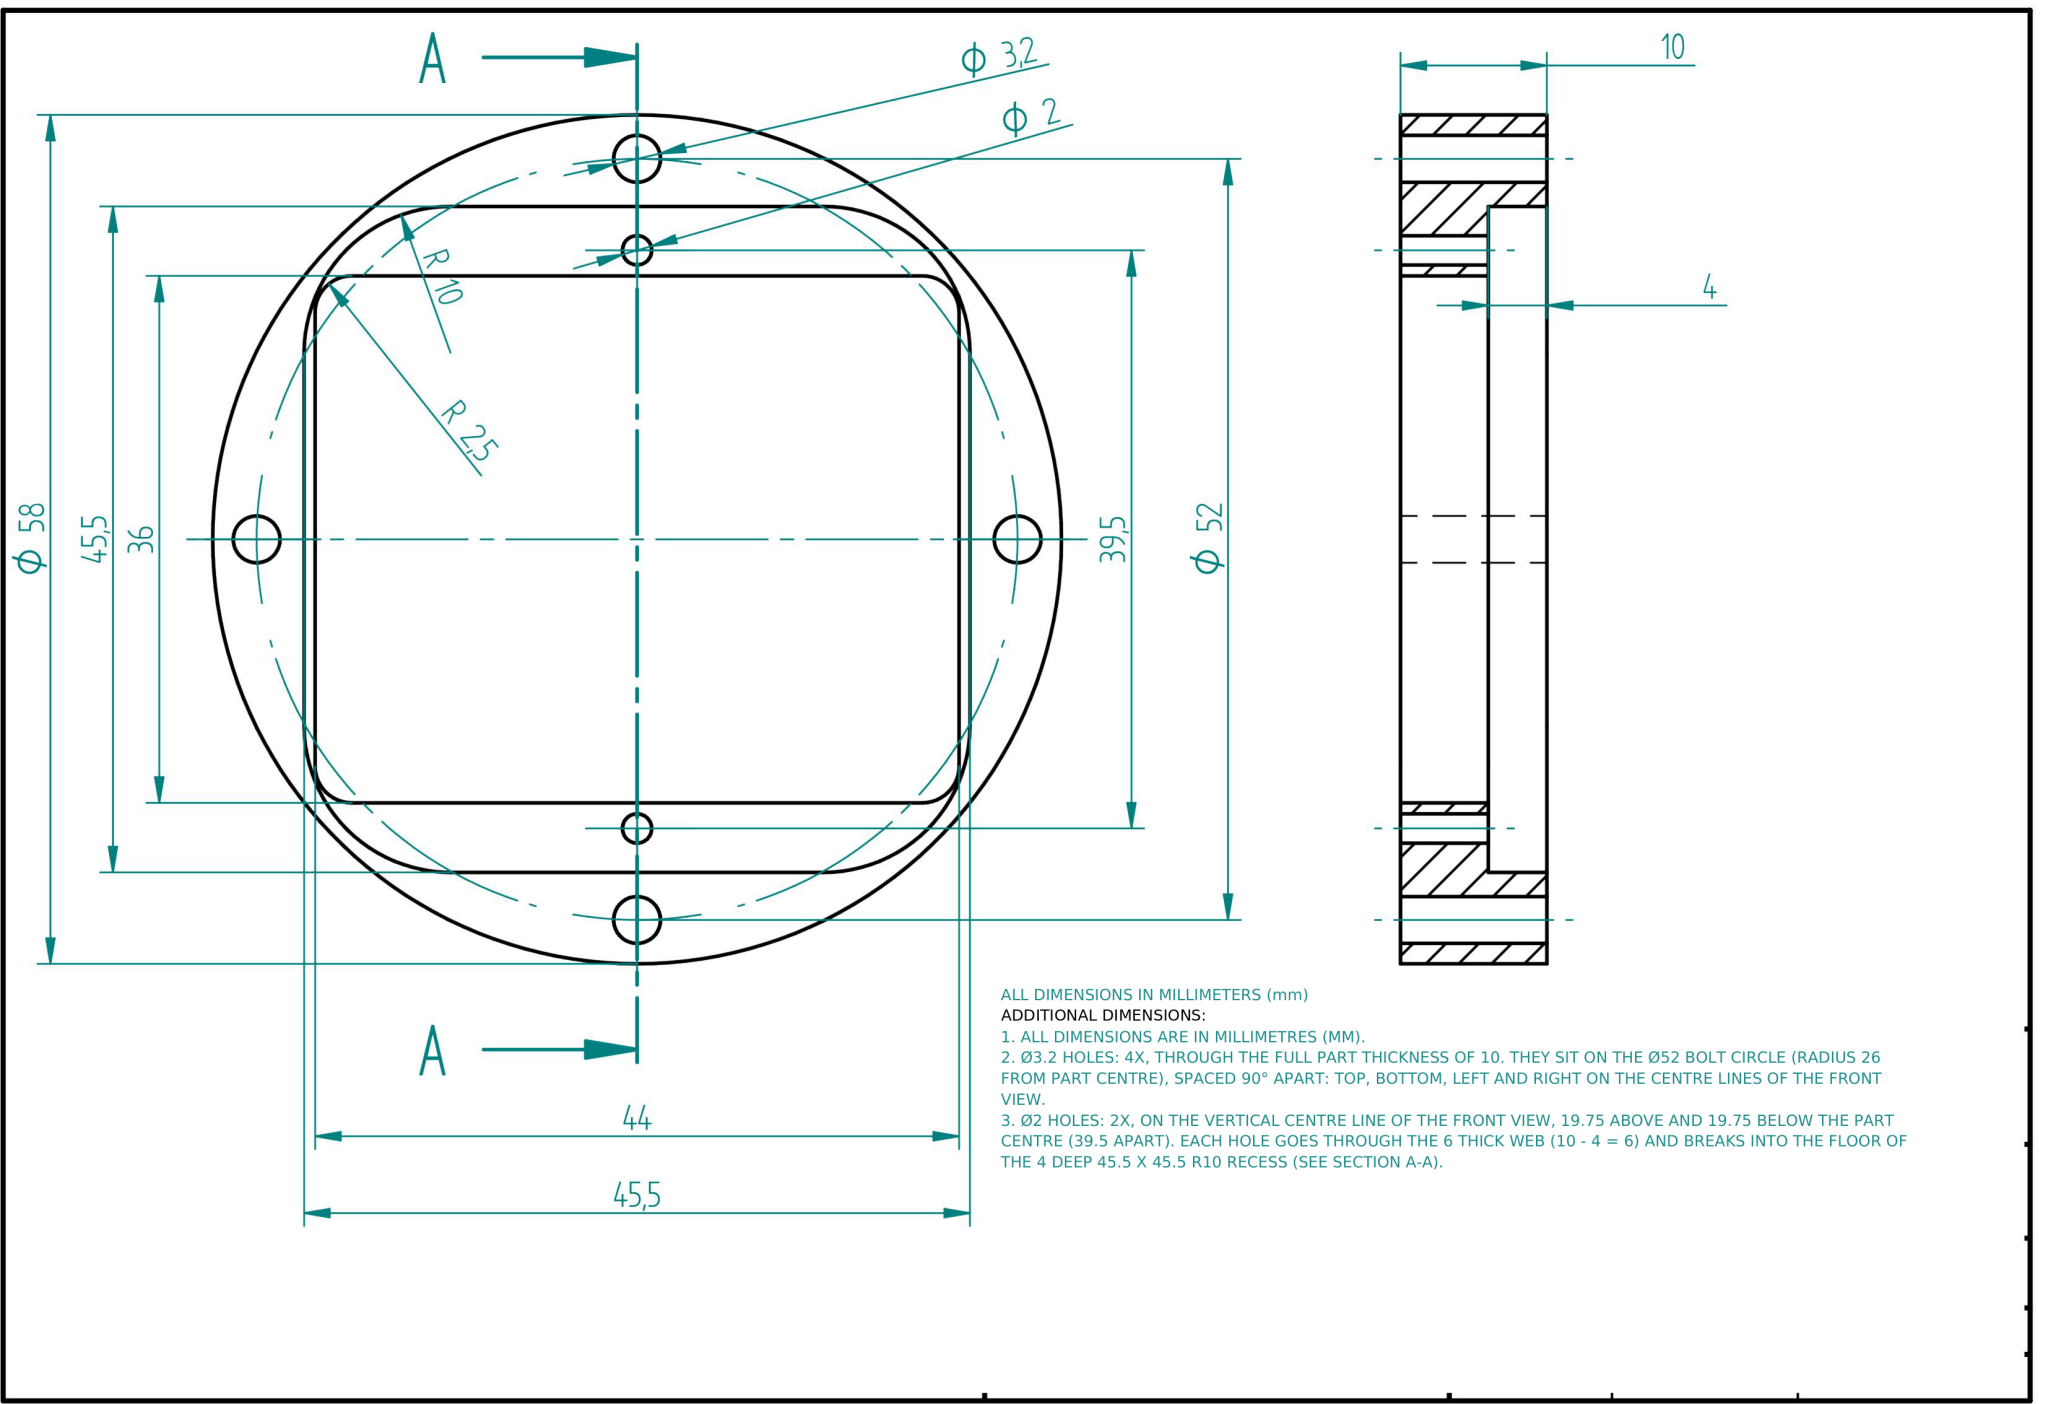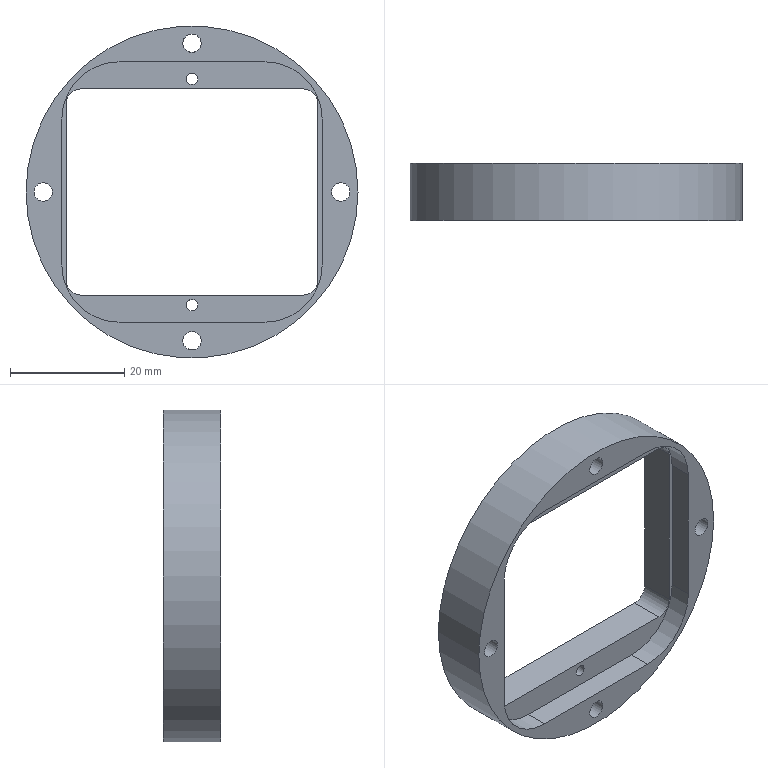Part | NX | mm | Triangular Flanged Gasket Ring | 1 solid | 26 faces | box 58 x 10 x 58 mm | volume 8652 mm3 | cylinder 15 | plane 11 | commonest cylinder face diameters 20 x4 5 x4 3.2 x4 2 x2 58 x1
STEP:
#1=COLOUR_RGB('',0.,0.698,0.);
#2=FILL_AREA_STYLE_COLOUR('',#1);
#3=FILL_AREA_STYLE('',(#2));
#4=SURFACE_STYLE_FILL_AREA(#3);
#5=SURFACE_SIDE_STYLE('',(#4));
#6=SURFACE_STYLE_USAGE(.BOTH.,#5);
#7=PRESENTATION_STYLE_ASSIGNMENT((#6));
#8=CARTESIAN_POINT('',(-26.,0.,1.6));
#9=VERTEX_POINT('',#8);
#10=CARTESIAN_POINT('',(-26.,0.,-0.));
#11=DIRECTION('',(0.,-1.,0.));
#12=DIRECTION('',(-0.,0.,1.));
#13=AXIS2_PLACEMENT_3D('',#10,#11,#12);
#14=CIRCLE('',#13,1.6);
#15=EDGE_CURVE('',#9,#9,#14,.T.);
#16=ORIENTED_EDGE('',*,*,#15,.F.);
#17=EDGE_LOOP('',(#16));
#18=FACE_BOUND('',#17,.T.);
#19=CARTESIAN_POINT('',(-1.6,0.,-26.));
#20=VERTEX_POINT('',#19);
#21=CARTESIAN_POINT('',(-0.,0.,-26.));
#22=DIRECTION('',(0.,-1.,0.));
#23=DIRECTION('',(-1.,0.,0.));
#24=AXIS2_PLACEMENT_3D('',#21,#22,#23);
#25=CIRCLE('',#24,1.6);
#26=EDGE_CURVE('',#20,#20,#25,.T.);
#27=ORIENTED_EDGE('',*,*,#26,.F.);
#28=EDGE_LOOP('',(#27));
#29=FACE_BOUND('',#28,.T.);
#30=CARTESIAN_POINT('',(26.,0.,-1.6));
#31=VERTEX_POINT('',#30);
#32=CARTESIAN_POINT('',(26.,0.,-0.));
#33=DIRECTION('',(0.,-1.,0.));
#34=DIRECTION('',(-0.,0.,-1.));
#35=AXIS2_PLACEMENT_3D('',#32,#33,#34);
#36=CIRCLE('',#35,1.6);
#37=EDGE_CURVE('',#31,#31,#36,.T.);
#38=ORIENTED_EDGE('',*,*,#37,.F.);
#39=EDGE_LOOP('',(#38));
#40=FACE_BOUND('',#39,.T.);
#41=CARTESIAN_POINT('',(1.6,0.,26.));
#42=VERTEX_POINT('',#41);
#43=CARTESIAN_POINT('',(0.,0.,26.));
#44=DIRECTION('',(0.,-1.,0.));
#45=DIRECTION('',(1.,0.,0.));
#46=AXIS2_PLACEMENT_3D('',#43,#44,#45);
#47=CIRCLE('',#46,1.6);
#48=EDGE_CURVE('',#42,#42,#47,.T.);
#49=ORIENTED_EDGE('',*,*,#48,.F.);
#50=EDGE_LOOP('',(#49));
#51=FACE_BOUND('',#50,.T.);
#52=CARTESIAN_POINT('',(29.,0.,0.));
#53=VERTEX_POINT('',#52);
#54=CARTESIAN_POINT('',(0.,0.,0.));
#55=DIRECTION('',(0.,1.,0.));
#56=DIRECTION('',(1.,0.,0.));
#57=AXIS2_PLACEMENT_3D('',#54,#55,#56);
#58=CIRCLE('',#57,29.);
#59=EDGE_CURVE('',#53,#53,#58,.T.);
#60=ORIENTED_EDGE('',*,*,#59,.F.);
#61=EDGE_LOOP('',(#60));
#62=FACE_OUTER_BOUND('',#61,.T.);
#63=CARTESIAN_POINT('',(22.75,0.,-12.75));
#64=VERTEX_POINT('',#63);
#65=CARTESIAN_POINT('',(12.75,0.,-22.75));
#66=VERTEX_POINT('',#65);
#67=CARTESIAN_POINT('',(12.75,0.,-12.75));
#68=DIRECTION('',(0.,1.,0.));
#69=DIRECTION('',(-1.,0.,0.));
#70=AXIS2_PLACEMENT_3D('',#67,#68,#69);
#71=CIRCLE('',#70,10.);
#72=EDGE_CURVE('',#64,#66,#71,.T.);
#73=ORIENTED_EDGE('',*,*,#72,.T.);
#74=CARTESIAN_POINT('',(-12.75,0.,-22.75));
#75=VERTEX_POINT('',#74);
#76=CARTESIAN_POINT('',(22.75,0.,-22.75));
#77=DIRECTION('',(-1.,0.,-0.));
#78=VECTOR('',#77,1000.);
#79=LINE('',#76,#78);
#80=EDGE_CURVE('',#66,#75,#79,.T.);
#81=ORIENTED_EDGE('',*,*,#80,.T.);
#82=CARTESIAN_POINT('',(-22.75,0.,-12.75));
#83=VERTEX_POINT('',#82);
#84=CARTESIAN_POINT('',(-12.75,0.,-12.75));
#85=DIRECTION('',(0.,1.,0.));
#86=DIRECTION('',(1.,0.,0.));
#87=AXIS2_PLACEMENT_3D('',#84,#85,#86);
#88=CIRCLE('',#87,10.);
#89=EDGE_CURVE('',#75,#83,#88,.T.);
#90=ORIENTED_EDGE('',*,*,#89,.T.);
#91=CARTESIAN_POINT('',(-22.75,0.,12.75));
#92=VERTEX_POINT('',#91);
#93=CARTESIAN_POINT('',(-22.75,0.,-22.75));
#94=DIRECTION('',(-0.,0.,1.));
#95=VECTOR('',#94,1000.);
#96=LINE('',#93,#95);
#97=EDGE_CURVE('',#83,#92,#96,.T.);
#98=ORIENTED_EDGE('',*,*,#97,.T.);
#99=CARTESIAN_POINT('',(-12.75,0.,22.75));
#100=VERTEX_POINT('',#99);
#101=CARTESIAN_POINT('',(-12.75,0.,12.75));
#102=DIRECTION('',(0.,1.,0.));
#103=DIRECTION('',(1.,0.,0.));
#104=AXIS2_PLACEMENT_3D('',#101,#102,#103);
#105=CIRCLE('',#104,10.);
#106=EDGE_CURVE('',#92,#100,#105,.T.);
#107=ORIENTED_EDGE('',*,*,#106,.T.);
#108=CARTESIAN_POINT('',(12.75,0.,22.75));
#109=VERTEX_POINT('',#108);
#110=CARTESIAN_POINT('',(-22.75,0.,22.75));
#111=DIRECTION('',(1.,0.,0.));
#112=VECTOR('',#111,1000.);
#113=LINE('',#110,#112);
#114=EDGE_CURVE('',#100,#109,#113,.T.);
#115=ORIENTED_EDGE('',*,*,#114,.T.);
#116=CARTESIAN_POINT('',(22.75,0.,12.75));
#117=VERTEX_POINT('',#116);
#118=CARTESIAN_POINT('',(12.75,0.,12.75));
#119=DIRECTION('',(0.,1.,0.));
#120=DIRECTION('',(-1.,0.,0.));
#121=AXIS2_PLACEMENT_3D('',#118,#119,#120);
#122=CIRCLE('',#121,10.);
#123=EDGE_CURVE('',#109,#117,#122,.T.);
#124=ORIENTED_EDGE('',*,*,#123,.T.);
#125=CARTESIAN_POINT('',(22.75,0.,22.75));
#126=DIRECTION('',(0.,0.,-1.));
#127=VECTOR('',#126,1000.);
#128=LINE('',#125,#127);
#129=EDGE_CURVE('',#117,#64,#128,.T.);
#130=ORIENTED_EDGE('',*,*,#129,.T.);
#131=EDGE_LOOP('',(#73,#81,#90,#98,#107,#115,#124,#130));
#132=FACE_BOUND('',#131,.T.);
#133=CARTESIAN_POINT('',(0.,0.,0.));
#134=DIRECTION('',(0.,1.,0.));
#135=DIRECTION('',(0.,0.,1.));
#136=AXIS2_PLACEMENT_3D('',#133,#134,#135);
#137=PLANE('',#136);
#138=ADVANCED_FACE('',(#18,#29,#40,#51,#62,#132),#137,.F.);
#139=STYLED_ITEM('',(#7),#138);
#140=COLOUR_RGB('',0.,0.698,0.);
#141=FILL_AREA_STYLE_COLOUR('',#140);
#142=FILL_AREA_STYLE('',(#141));
#143=SURFACE_STYLE_FILL_AREA(#142);
#144=SURFACE_SIDE_STYLE('',(#143));
#145=SURFACE_STYLE_USAGE(.BOTH.,#144);
#146=PRESENTATION_STYLE_ASSIGNMENT((#145));
#147=ORIENTED_EDGE('',*,*,#80,.F.);
#148=CARTESIAN_POINT('',(12.75,4.,-22.75));
#149=VERTEX_POINT('',#148);
#150=CARTESIAN_POINT('',(12.75,4.,-22.75));
#151=DIRECTION('',(0.,-1.,0.));
#152=VECTOR('',#151,1000.);
#153=LINE('',#150,#152);
#154=EDGE_CURVE('',#149,#66,#153,.T.);
#155=ORIENTED_EDGE('',*,*,#154,.F.);
#156=CARTESIAN_POINT('',(-12.75,4.,-22.75));
#157=VERTEX_POINT('',#156);
#158=CARTESIAN_POINT('',(22.75,4.,-22.75));
#159=DIRECTION('',(-1.,0.,-0.));
#160=VECTOR('',#159,1000.);
#161=LINE('',#158,#160);
#162=EDGE_CURVE('',#149,#157,#161,.T.);
#163=ORIENTED_EDGE('',*,*,#162,.T.);
#164=CARTESIAN_POINT('',(-12.75,4.,-22.75));
#165=DIRECTION('',(0.,-1.,0.));
#166=VECTOR('',#165,1000.);
#167=LINE('',#164,#166);
#168=EDGE_CURVE('',#157,#75,#167,.T.);
#169=ORIENTED_EDGE('',*,*,#168,.T.);
#170=EDGE_LOOP('',(#147,#155,#163,#169));
#171=FACE_OUTER_BOUND('',#170,.T.);
#172=CARTESIAN_POINT('',(22.75,4.,-22.75));
#173=DIRECTION('',(-0.,0.,1.));
#174=DIRECTION('',(1.,0.,0.));
#175=AXIS2_PLACEMENT_3D('',#172,#173,#174);
#176=PLANE('',#175);
#177=ADVANCED_FACE('',(#171),#176,.T.);
#178=STYLED_ITEM('',(#146),#177);
#179=COLOUR_RGB('',0.,0.698,0.);
#180=FILL_AREA_STYLE_COLOUR('',#179);
#181=FILL_AREA_STYLE('',(#180));
#182=SURFACE_STYLE_FILL_AREA(#181);
#183=SURFACE_SIDE_STYLE('',(#182));
#184=SURFACE_STYLE_USAGE(.BOTH.,#183);
#185=PRESENTATION_STYLE_ASSIGNMENT((#184));
#186=CARTESIAN_POINT('',(19.5,4.,-18.));
#187=VERTEX_POINT('',#186);
#188=CARTESIAN_POINT('',(-19.5,4.,-18.));
#189=VERTEX_POINT('',#188);
#190=CARTESIAN_POINT('',(22.,4.,-18.));
#191=DIRECTION('',(-1.,0.,0.));
#192=VECTOR('',#191,1000.);
#193=LINE('',#190,#192);
#194=EDGE_CURVE('',#187,#189,#193,.T.);
#195=ORIENTED_EDGE('',*,*,#194,.F.);
#196=CARTESIAN_POINT('',(19.5,10.,-18.));
#197=VERTEX_POINT('',#196);
#198=CARTESIAN_POINT('',(19.5,84.,-18.));
#199=DIRECTION('',(0.,-1.,0.));
#200=VECTOR('',#199,1000.);
#201=LINE('',#198,#200);
#202=EDGE_CURVE('',#197,#187,#201,.T.);
#203=ORIENTED_EDGE('',*,*,#202,.F.);
#204=CARTESIAN_POINT('',(-19.5,10.,-18.));
#205=VERTEX_POINT('',#204);
#206=CARTESIAN_POINT('',(0.,10.,-18.));
#207=DIRECTION('',(1.,0.,0.));
#208=VECTOR('',#207,1000.);
#209=LINE('',#206,#208);
#210=EDGE_CURVE('',#205,#197,#209,.T.);
#211=ORIENTED_EDGE('',*,*,#210,.F.);
#212=CARTESIAN_POINT('',(-19.5,84.,-18.));
#213=DIRECTION('',(0.,-1.,0.));
#214=VECTOR('',#213,1000.);
#215=LINE('',#212,#214);
#216=EDGE_CURVE('',#205,#189,#215,.T.);
#217=ORIENTED_EDGE('',*,*,#216,.T.);
#218=EDGE_LOOP('',(#195,#203,#211,#217));
#219=FACE_OUTER_BOUND('',#218,.T.);
#220=CARTESIAN_POINT('',(22.,84.,-18.));
#221=DIRECTION('',(0.,0.,1.));
#222=DIRECTION('',(1.,0.,0.));
#223=AXIS2_PLACEMENT_3D('',#220,#221,#222);
#224=PLANE('',#223);
#225=ADVANCED_FACE('',(#219),#224,.T.);
#226=STYLED_ITEM('',(#185),#225);
#227=COLOUR_RGB('',0.,0.698,0.);
#228=FILL_AREA_STYLE_COLOUR('',#227);
#229=FILL_AREA_STYLE('',(#228));
#230=SURFACE_STYLE_FILL_AREA(#229);
#231=SURFACE_SIDE_STYLE('',(#230));
#232=SURFACE_STYLE_USAGE(.BOTH.,#231);
#233=PRESENTATION_STYLE_ASSIGNMENT((#232));
#234=CARTESIAN_POINT('',(0.,10.,-18.75));
#235=VERTEX_POINT('',#234);
#236=CARTESIAN_POINT('',(0.,10.,-19.75));
#237=DIRECTION('',(0.,1.,0.));
#238=DIRECTION('',(0.,0.,1.));
#239=AXIS2_PLACEMENT_3D('',#236,#237,#238);
#240=CIRCLE('',#239,1.);
#241=EDGE_CURVE('',#235,#235,#240,.T.);
#242=ORIENTED_EDGE('',*,*,#241,.F.);
#243=EDGE_LOOP('',(#242));
#244=FACE_BOUND('',#243,.T.);
#245=CARTESIAN_POINT('',(0.,10.,20.75));
#246=VERTEX_POINT('',#245);
#247=CARTESIAN_POINT('',(0.,10.,19.75));
#248=DIRECTION('',(0.,1.,0.));
#249=DIRECTION('',(0.,0.,1.));
#250=AXIS2_PLACEMENT_3D('',#247,#248,#249);
#251=CIRCLE('',#250,1.);
#252=EDGE_CURVE('',#246,#246,#251,.T.);
#253=ORIENTED_EDGE('',*,*,#252,.F.);
#254=EDGE_LOOP('',(#253));
#255=FACE_BOUND('',#254,.T.);
#256=CARTESIAN_POINT('',(-26.,10.,1.6));
#257=VERTEX_POINT('',#256);
#258=CARTESIAN_POINT('',(-26.,10.,-0.));
#259=DIRECTION('',(0.,1.,0.));
#260=DIRECTION('',(0.,0.,1.));
#261=AXIS2_PLACEMENT_3D('',#258,#259,#260);
#262=CIRCLE('',#261,1.6);
#263=EDGE_CURVE('',#257,#257,#262,.T.);
#264=ORIENTED_EDGE('',*,*,#263,.F.);
#265=EDGE_LOOP('',(#264));
#266=FACE_BOUND('',#265,.T.);
#267=CARTESIAN_POINT('',(-0.,10.,-24.4));
#268=VERTEX_POINT('',#267);
#269=CARTESIAN_POINT('',(-0.,10.,-26.));
#270=DIRECTION('',(0.,1.,0.));
#271=DIRECTION('',(0.,0.,1.));
#272=AXIS2_PLACEMENT_3D('',#269,#270,#271);
#273=CIRCLE('',#272,1.6);
#274=EDGE_CURVE('',#268,#268,#273,.T.);
#275=ORIENTED_EDGE('',*,*,#274,.F.);
#276=EDGE_LOOP('',(#275));
#277=FACE_BOUND('',#276,.T.);
#278=CARTESIAN_POINT('',(26.,10.,1.6));
#279=VERTEX_POINT('',#278);
#280=CARTESIAN_POINT('',(26.,10.,-0.));
#281=DIRECTION('',(0.,1.,0.));
#282=DIRECTION('',(0.,0.,1.));
#283=AXIS2_PLACEMENT_3D('',#280,#281,#282);
#284=CIRCLE('',#283,1.6);
#285=EDGE_CURVE('',#279,#279,#284,.T.);
#286=ORIENTED_EDGE('',*,*,#285,.F.);
#287=EDGE_LOOP('',(#286));
#288=FACE_BOUND('',#287,.T.);
#289=CARTESIAN_POINT('',(0.,10.,27.6));
#290=VERTEX_POINT('',#289);
#291=CARTESIAN_POINT('',(0.,10.,26.));
#292=DIRECTION('',(0.,1.,0.));
#293=DIRECTION('',(0.,0.,1.));
#294=AXIS2_PLACEMENT_3D('',#291,#292,#293);
#295=CIRCLE('',#294,1.6);
#296=EDGE_CURVE('',#290,#290,#295,.T.);
#297=ORIENTED_EDGE('',*,*,#296,.F.);
#298=EDGE_LOOP('',(#297));
#299=FACE_BOUND('',#298,.T.);
#300=CARTESIAN_POINT('',(29.,10.,0.));
#301=VERTEX_POINT('',#300);
#302=CARTESIAN_POINT('',(0.,10.,0.));
#303=DIRECTION('',(0.,1.,0.));
#304=DIRECTION('',(1.,0.,0.));
#305=AXIS2_PLACEMENT_3D('',#302,#303,#304);
#306=CIRCLE('',#305,29.);
#307=EDGE_CURVE('',#301,#301,#306,.T.);
#308=ORIENTED_EDGE('',*,*,#307,.T.);
#309=EDGE_LOOP('',(#308));
#310=FACE_OUTER_BOUND('',#309,.T.);
#311=CARTESIAN_POINT('',(19.5,10.,18.));
#312=VERTEX_POINT('',#311);
#313=CARTESIAN_POINT('',(-19.5,10.,18.));
#314=VERTEX_POINT('',#313);
#315=CARTESIAN_POINT('',(0.,10.,18.));
#316=DIRECTION('',(-1.,0.,0.));
#317=VECTOR('',#316,1000.);
#318=LINE('',#315,#317);
#319=EDGE_CURVE('',#312,#314,#318,.T.);
#320=ORIENTED_EDGE('',*,*,#319,.T.);
#321=CARTESIAN_POINT('',(-22.,10.,15.5));
#322=VERTEX_POINT('',#321);
#323=CARTESIAN_POINT('',(-19.5,10.,15.5));
#324=DIRECTION('',(0.,1.,0.));
#325=DIRECTION('',(0.,0.,1.));
#326=AXIS2_PLACEMENT_3D('',#323,#324,#325);
#327=CIRCLE('',#326,2.5);
#328=EDGE_CURVE('',#314,#322,#327,.F.);
#329=ORIENTED_EDGE('',*,*,#328,.T.);
#330=CARTESIAN_POINT('',(-22.,10.,-15.5));
#331=VERTEX_POINT('',#330);
#332=CARTESIAN_POINT('',(-22.,10.,0.));
#333=DIRECTION('',(0.,0.,-1.));
#334=VECTOR('',#333,1000.);
#335=LINE('',#332,#334);
#336=EDGE_CURVE('',#322,#331,#335,.T.);
#337=ORIENTED_EDGE('',*,*,#336,.T.);
#338=CARTESIAN_POINT('',(-19.5,10.,-15.5));
#339=DIRECTION('',(0.,1.,0.));
#340=DIRECTION('',(0.,0.,1.));
#341=AXIS2_PLACEMENT_3D('',#338,#339,#340);
#342=CIRCLE('',#341,2.5);
#343=EDGE_CURVE('',#331,#205,#342,.F.);
#344=ORIENTED_EDGE('',*,*,#343,.T.);
#345=ORIENTED_EDGE('',*,*,#210,.T.);
#346=CARTESIAN_POINT('',(22.,10.,-15.5));
#347=VERTEX_POINT('',#346);
#348=CARTESIAN_POINT('',(19.5,10.,-15.5));
#349=DIRECTION('',(0.,1.,0.));
#350=DIRECTION('',(0.,0.,1.));
#351=AXIS2_PLACEMENT_3D('',#348,#349,#350);
#352=CIRCLE('',#351,2.5);
#353=EDGE_CURVE('',#197,#347,#352,.F.);
#354=ORIENTED_EDGE('',*,*,#353,.T.);
#355=CARTESIAN_POINT('',(22.,10.,15.5));
#356=VERTEX_POINT('',#355);
#357=CARTESIAN_POINT('',(22.,10.,0.));
#358=DIRECTION('',(0.,0.,1.));
#359=VECTOR('',#358,1000.);
#360=LINE('',#357,#359);
#361=EDGE_CURVE('',#347,#356,#360,.T.);
#362=ORIENTED_EDGE('',*,*,#361,.T.);
#363=CARTESIAN_POINT('',(19.5,10.,15.5));
#364=DIRECTION('',(0.,1.,0.));
#365=DIRECTION('',(0.,0.,1.));
#366=AXIS2_PLACEMENT_3D('',#363,#364,#365);
#367=CIRCLE('',#366,2.5);
#368=EDGE_CURVE('',#356,#312,#367,.F.);
#369=ORIENTED_EDGE('',*,*,#368,.T.);
#370=EDGE_LOOP('',(#320,#329,#337,#344,#345,#354,#362,#369));
#371=FACE_BOUND('',#370,.T.);
#372=CARTESIAN_POINT('',(0.,10.,0.));
#373=DIRECTION('',(0.,1.,0.));
#374=DIRECTION('',(0.,0.,1.));
#375=AXIS2_PLACEMENT_3D('',#372,#373,#374);
#376=PLANE('',#375);
#377=ADVANCED_FACE('',(#244,#255,#266,#277,#288,#299,#310,#371),#376,.T.);
#378=STYLED_ITEM('',(#233),#377);
#379=COLOUR_RGB('',0.,0.698,0.);
#380=FILL_AREA_STYLE_COLOUR('',#379);
#381=FILL_AREA_STYLE('',(#380));
#382=SURFACE_STYLE_FILL_AREA(#381);
#383=SURFACE_SIDE_STYLE('',(#382));
#384=SURFACE_STYLE_USAGE(.BOTH.,#383);
#385=PRESENTATION_STYLE_ASSIGNMENT((#384));
#386=ORIENTED_EDGE('',*,*,#129,.F.);
#387=CARTESIAN_POINT('',(22.75,4.,12.75));
#388=VERTEX_POINT('',#387);
#389=CARTESIAN_POINT('',(22.75,4.,12.75));
#390=DIRECTION('',(0.,-1.,0.));
#391=VECTOR('',#390,1000.);
#392=LINE('',#389,#391);
#393=EDGE_CURVE('',#388,#117,#392,.T.);
#394=ORIENTED_EDGE('',*,*,#393,.F.);
#395=CARTESIAN_POINT('',(22.75,4.,-12.75));
#396=VERTEX_POINT('',#395);
#397=CARTESIAN_POINT('',(22.75,4.,22.75));
#398=DIRECTION('',(0.,0.,-1.));
#399=VECTOR('',#398,1000.);
#400=LINE('',#397,#399);
#401=EDGE_CURVE('',#388,#396,#400,.T.);
#402=ORIENTED_EDGE('',*,*,#401,.T.);
#403=CARTESIAN_POINT('',(22.75,4.,-12.75));
#404=DIRECTION('',(0.,-1.,0.));
#405=VECTOR('',#404,1000.);
#406=LINE('',#403,#405);
#407=EDGE_CURVE('',#396,#64,#406,.T.);
#408=ORIENTED_EDGE('',*,*,#407,.T.);
#409=EDGE_LOOP('',(#386,#394,#402,#408));
#410=FACE_OUTER_BOUND('',#409,.T.);
#411=CARTESIAN_POINT('',(22.75,4.,22.75));
#412=DIRECTION('',(-1.,0.,-0.));
#413=DIRECTION('',(-0.,0.,1.));
#414=AXIS2_PLACEMENT_3D('',#411,#412,#413);
#415=PLANE('',#414);
#416=ADVANCED_FACE('',(#410),#415,.T.);
#417=STYLED_ITEM('',(#385),#416);
#418=COLOUR_RGB('',0.,0.698,0.);
#419=FILL_AREA_STYLE_COLOUR('',#418);
#420=FILL_AREA_STYLE('',(#419));
#421=SURFACE_STYLE_FILL_AREA(#420);
#422=SURFACE_SIDE_STYLE('',(#421));
#423=SURFACE_STYLE_USAGE(.BOTH.,#422);
#424=PRESENTATION_STYLE_ASSIGNMENT((#423));
#425=ORIENTED_EDGE('',*,*,#72,.F.);
#426=ORIENTED_EDGE('',*,*,#407,.F.);
#427=CARTESIAN_POINT('',(12.75,4.,-12.75));
#428=DIRECTION('',(0.,1.,0.));
#429=DIRECTION('',(-1.,0.,0.));
#430=AXIS2_PLACEMENT_3D('',#427,#428,#429);
#431=CIRCLE('',#430,10.);
#432=EDGE_CURVE('',#396,#149,#431,.T.);
#433=ORIENTED_EDGE('',*,*,#432,.T.);
#434=ORIENTED_EDGE('',*,*,#154,.T.);
#435=EDGE_LOOP('',(#425,#426,#433,#434));
#436=FACE_OUTER_BOUND('',#435,.T.);
#437=CARTESIAN_POINT('',(12.75,4.,-12.75));
#438=DIRECTION('',(0.,1.,0.));
#439=DIRECTION('',(0.,0.,-1.));
#440=AXIS2_PLACEMENT_3D('',#437,#438,#439);
#441=CYLINDRICAL_SURFACE('',#440,10.);
#442=ADVANCED_FACE('',(#436),#441,.F.);
#443=STYLED_ITEM('',(#424),#442);
#444=COLOUR_RGB('',0.,0.698,0.);
#445=FILL_AREA_STYLE_COLOUR('',#444);
#446=FILL_AREA_STYLE('',(#445));
#447=SURFACE_STYLE_FILL_AREA(#446);
#448=SURFACE_SIDE_STYLE('',(#447));
#449=SURFACE_STYLE_USAGE(.BOTH.,#448);
#450=PRESENTATION_STYLE_ASSIGNMENT((#449));
#451=ORIENTED_EDGE('',*,*,#48,.T.);
#452=EDGE_LOOP('',(#451));
#453=FACE_OUTER_BOUND('',#452,.T.);
#454=ORIENTED_EDGE('',*,*,#296,.T.);
#455=EDGE_LOOP('',(#454));
#456=FACE_OUTER_BOUND('',#455,.T.);
#457=CARTESIAN_POINT('',(0.,82.632,26.));
#458=DIRECTION('',(0.,1.,0.));
#459=DIRECTION('',(0.,0.,-1.));
#460=AXIS2_PLACEMENT_3D('',#457,#458,#459);
#461=CYLINDRICAL_SURFACE('',#460,1.6);
#462=ADVANCED_FACE('',(#453,#456),#461,.F.);
#463=STYLED_ITEM('',(#450),#462);
#464=COLOUR_RGB('',0.,0.698,0.);
#465=FILL_AREA_STYLE_COLOUR('',#464);
#466=FILL_AREA_STYLE('',(#465));
#467=SURFACE_STYLE_FILL_AREA(#466);
#468=SURFACE_SIDE_STYLE('',(#467));
#469=SURFACE_STYLE_USAGE(.BOTH.,#468);
#470=PRESENTATION_STYLE_ASSIGNMENT((#469));
#471=ORIENTED_EDGE('',*,*,#97,.F.);
#472=CARTESIAN_POINT('',(-22.75,4.,-12.75));
#473=VERTEX_POINT('',#472);
#474=CARTESIAN_POINT('',(-22.75,4.,-12.75));
#475=DIRECTION('',(0.,-1.,0.));
#476=VECTOR('',#475,1000.);
#477=LINE('',#474,#476);
#478=EDGE_CURVE('',#473,#83,#477,.T.);
#479=ORIENTED_EDGE('',*,*,#478,.F.);
#480=CARTESIAN_POINT('',(-22.75,4.,12.75));
#481=VERTEX_POINT('',#480);
#482=CARTESIAN_POINT('',(-22.75,4.,-22.75));
#483=DIRECTION('',(-0.,0.,1.));
#484=VECTOR('',#483,1000.);
#485=LINE('',#482,#484);
#486=EDGE_CURVE('',#473,#481,#485,.T.);
#487=ORIENTED_EDGE('',*,*,#486,.T.);
#488=CARTESIAN_POINT('',(-22.75,4.,12.75));
#489=DIRECTION('',(0.,-1.,0.));
#490=VECTOR('',#489,1000.);
#491=LINE('',#488,#490);
#492=EDGE_CURVE('',#481,#92,#491,.T.);
#493=ORIENTED_EDGE('',*,*,#492,.T.);
#494=EDGE_LOOP('',(#471,#479,#487,#493));
#495=FACE_OUTER_BOUND('',#494,.T.);
#496=CARTESIAN_POINT('',(-22.75,4.,-22.75));
#497=DIRECTION('',(1.,0.,0.));
#498=DIRECTION('',(0.,0.,-1.));
#499=AXIS2_PLACEMENT_3D('',#496,#497,#498);
#500=PLANE('',#499);
#501=ADVANCED_FACE('',(#495),#500,.T.);
#502=STYLED_ITEM('',(#470),#501);
#503=COLOUR_RGB('',0.,0.698,0.);
#504=FILL_AREA_STYLE_COLOUR('',#503);
#505=FILL_AREA_STYLE('',(#504));
#506=SURFACE_STYLE_FILL_AREA(#505);
#507=SURFACE_SIDE_STYLE('',(#506));
#508=SURFACE_STYLE_USAGE(.BOTH.,#507);
#509=PRESENTATION_STYLE_ASSIGNMENT((#508));
#510=CARTESIAN_POINT('',(19.5,4.,18.));
#511=VERTEX_POINT('',#510);
#512=CARTESIAN_POINT('',(22.,4.,15.5));
#513=VERTEX_POINT('',#512);
#514=CARTESIAN_POINT('',(19.5,4.,15.5));
#515=DIRECTION('',(0.,1.,0.));
#516=DIRECTION('',(0.,0.,1.));
#517=AXIS2_PLACEMENT_3D('',#514,#515,#516);
#518=CIRCLE('',#517,2.5);
#519=EDGE_CURVE('',#511,#513,#518,.T.);
#520=ORIENTED_EDGE('',*,*,#519,.F.);
#521=CARTESIAN_POINT('',(19.5,84.,18.));
#522=DIRECTION('',(0.,-1.,0.));
#523=VECTOR('',#522,1000.);
#524=LINE('',#521,#523);
#525=EDGE_CURVE('',#312,#511,#524,.T.);
#526=ORIENTED_EDGE('',*,*,#525,.F.);
#527=ORIENTED_EDGE('',*,*,#368,.F.);
#528=CARTESIAN_POINT('',(22.,84.,15.5));
#529=DIRECTION('',(0.,-1.,0.));
#530=VECTOR('',#529,1000.);
#531=LINE('',#528,#530);
#532=EDGE_CURVE('',#356,#513,#531,.T.);
#533=ORIENTED_EDGE('',*,*,#532,.T.);
#534=EDGE_LOOP('',(#520,#526,#527,#533));
#535=FACE_OUTER_BOUND('',#534,.T.);
#536=CARTESIAN_POINT('',(19.5,84.,15.5));
#537=DIRECTION('',(0.,1.,0.));
#538=DIRECTION('',(0.,0.,-1.));
#539=AXIS2_PLACEMENT_3D('',#536,#537,#538);
#540=CYLINDRICAL_SURFACE('',#539,2.5);
#541=ADVANCED_FACE('',(#535),#540,.F.);
#542=STYLED_ITEM('',(#509),#541);
#543=COLOUR_RGB('',0.,0.698,0.);
#544=FILL_AREA_STYLE_COLOUR('',#543);
#545=FILL_AREA_STYLE('',(#544));
#546=SURFACE_STYLE_FILL_AREA(#545);
#547=SURFACE_SIDE_STYLE('',(#546));
#548=SURFACE_STYLE_USAGE(.BOTH.,#547);
#549=PRESENTATION_STYLE_ASSIGNMENT((#548));
#550=CARTESIAN_POINT('',(-22.,4.,-15.5));
#551=VERTEX_POINT('',#550);
#552=CARTESIAN_POINT('',(-19.5,4.,-15.5));
#553=DIRECTION('',(0.,1.,0.));
#554=DIRECTION('',(0.,0.,1.));
#555=AXIS2_PLACEMENT_3D('',#552,#553,#554);
#556=CIRCLE('',#555,2.5);
#557=EDGE_CURVE('',#189,#551,#556,.T.);
#558=ORIENTED_EDGE('',*,*,#557,.F.);
#559=ORIENTED_EDGE('',*,*,#216,.F.);
#560=ORIENTED_EDGE('',*,*,#343,.F.);
#561=CARTESIAN_POINT('',(-22.,84.,-15.5));
#562=DIRECTION('',(0.,-1.,0.));
#563=VECTOR('',#562,1000.);
#564=LINE('',#561,#563);
#565=EDGE_CURVE('',#331,#551,#564,.T.);
#566=ORIENTED_EDGE('',*,*,#565,.T.);
#567=EDGE_LOOP('',(#558,#559,#560,#566));
#568=FACE_OUTER_BOUND('',#567,.T.);
#569=CARTESIAN_POINT('',(-19.5,84.,-15.5));
#570=DIRECTION('',(0.,1.,0.));
#571=DIRECTION('',(0.,0.,-1.));
#572=AXIS2_PLACEMENT_3D('',#569,#570,#571);
#573=CYLINDRICAL_SURFACE('',#572,2.5);
#574=ADVANCED_FACE('',(#568),#573,.F.);
#575=STYLED_ITEM('',(#549),#574);
#576=COLOUR_RGB('',0.,0.698,0.);
#577=FILL_AREA_STYLE_COLOUR('',#576);
#578=FILL_AREA_STYLE('',(#577));
#579=SURFACE_STYLE_FILL_AREA(#578);
#580=SURFACE_SIDE_STYLE('',(#579));
#581=SURFACE_STYLE_USAGE(.BOTH.,#580);
#582=PRESENTATION_STYLE_ASSIGNMENT((#581));
#583=ORIENTED_EDGE('',*,*,#307,.F.);
#584=EDGE_LOOP('',(#583));
#585=FACE_OUTER_BOUND('',#584,.T.);
#586=ORIENTED_EDGE('',*,*,#59,.T.);
#587=EDGE_LOOP('',(#586));
#588=FACE_OUTER_BOUND('',#587,.T.);
#589=CARTESIAN_POINT('',(0.,10.,0.));
#590=DIRECTION('',(0.,1.,0.));
#591=DIRECTION('',(0.,0.,-1.));
#592=AXIS2_PLACEMENT_3D('',#589,#590,#591);
#593=CYLINDRICAL_SURFACE('',#592,29.);
#594=ADVANCED_FACE('',(#585,#588),#593,.T.);
#595=STYLED_ITEM('',(#582),#594);
#596=COLOUR_RGB('',0.,0.698,0.);
#597=FILL_AREA_STYLE_COLOUR('',#596);
#598=FILL_AREA_STYLE('',(#597));
#599=SURFACE_STYLE_FILL_AREA(#598);
#600=SURFACE_SIDE_STYLE('',(#599));
#601=SURFACE_STYLE_USAGE(.BOTH.,#600);
#602=PRESENTATION_STYLE_ASSIGNMENT((#601));
#603=ORIENTED_EDGE('',*,*,#26,.T.);
#604=EDGE_LOOP('',(#603));
#605=FACE_OUTER_BOUND('',#604,.T.);
#606=ORIENTED_EDGE('',*,*,#274,.T.);
#607=EDGE_LOOP('',(#606));
#608=FACE_OUTER_BOUND('',#607,.T.);
#609=CARTESIAN_POINT('',(-0.,82.632,-26.));
#610=DIRECTION('',(0.,1.,0.));
#611=DIRECTION('',(0.,0.,-1.));
#612=AXIS2_PLACEMENT_3D('',#609,#610,#611);
#613=CYLINDRICAL_SURFACE('',#612,1.6);
#614=ADVANCED_FACE('',(#605,#608),#613,.F.);
#615=STYLED_ITEM('',(#602),#614);
#616=COLOUR_RGB('',0.,0.698,0.);
#617=FILL_AREA_STYLE_COLOUR('',#616);
#618=FILL_AREA_STYLE('',(#617));
#619=SURFACE_STYLE_FILL_AREA(#618);
#620=SURFACE_SIDE_STYLE('',(#619));
#621=SURFACE_STYLE_USAGE(.BOTH.,#620);
#622=PRESENTATION_STYLE_ASSIGNMENT((#621));
#623=ORIENTED_EDGE('',*,*,#106,.F.);
#624=ORIENTED_EDGE('',*,*,#492,.F.);
#625=CARTESIAN_POINT('',(-12.75,4.,22.75));
#626=VERTEX_POINT('',#625);
#627=CARTESIAN_POINT('',(-12.75,4.,12.75));
#628=DIRECTION('',(0.,1.,0.));
#629=DIRECTION('',(1.,0.,0.));
#630=AXIS2_PLACEMENT_3D('',#627,#628,#629);
#631=CIRCLE('',#630,10.);
#632=EDGE_CURVE('',#481,#626,#631,.T.);
#633=ORIENTED_EDGE('',*,*,#632,.T.);
#634=CARTESIAN_POINT('',(-12.75,4.,22.75));
#635=DIRECTION('',(0.,-1.,0.));
#636=VECTOR('',#635,1000.);
#637=LINE('',#634,#636);
#638=EDGE_CURVE('',#626,#100,#637,.T.);
#639=ORIENTED_EDGE('',*,*,#638,.T.);
#640=EDGE_LOOP('',(#623,#624,#633,#639));
#641=FACE_OUTER_BOUND('',#640,.T.);
#642=CARTESIAN_POINT('',(-12.75,4.,12.75));
#643=DIRECTION('',(0.,1.,0.));
#644=DIRECTION('',(0.,0.,-1.));
#645=AXIS2_PLACEMENT_3D('',#642,#643,#644);
#646=CYLINDRICAL_SURFACE('',#645,10.);
#647=ADVANCED_FACE('',(#641),#646,.F.);
#648=STYLED_ITEM('',(#622),#647);
#649=COLOUR_RGB('',0.,0.698,0.);
#650=FILL_AREA_STYLE_COLOUR('',#649);
#651=FILL_AREA_STYLE('',(#650));
#652=SURFACE_STYLE_FILL_AREA(#651);
#653=SURFACE_SIDE_STYLE('',(#652));
#654=SURFACE_STYLE_USAGE(.BOTH.,#653);
#655=PRESENTATION_STYLE_ASSIGNMENT((#654));
#656=ORIENTED_EDGE('',*,*,#114,.F.);
#657=ORIENTED_EDGE('',*,*,#638,.F.);
#658=CARTESIAN_POINT('',(12.75,4.,22.75));
#659=VERTEX_POINT('',#658);
#660=CARTESIAN_POINT('',(-22.75,4.,22.75));
#661=DIRECTION('',(1.,0.,0.));
#662=VECTOR('',#661,1000.);
#663=LINE('',#660,#662);
#664=EDGE_CURVE('',#626,#659,#663,.T.);
#665=ORIENTED_EDGE('',*,*,#664,.T.);
#666=CARTESIAN_POINT('',(12.75,4.,22.75));
#667=DIRECTION('',(0.,-1.,0.));
#668=VECTOR('',#667,1000.);
#669=LINE('',#666,#668);
#670=EDGE_CURVE('',#659,#109,#669,.T.);
#671=ORIENTED_EDGE('',*,*,#670,.T.);
#672=EDGE_LOOP('',(#656,#657,#665,#671));
#673=FACE_OUTER_BOUND('',#672,.T.);
#674=CARTESIAN_POINT('',(-22.75,4.,22.75));
#675=DIRECTION('',(0.,0.,-1.));
#676=DIRECTION('',(-1.,0.,-0.));
#677=AXIS2_PLACEMENT_3D('',#674,#675,#676);
#678=PLANE('',#677);
#679=ADVANCED_FACE('',(#673),#678,.T.);
#680=STYLED_ITEM('',(#655),#679);
#681=COLOUR_RGB('',0.,0.698,0.);
#682=FILL_AREA_STYLE_COLOUR('',#681);
#683=FILL_AREA_STYLE('',(#682));
#684=SURFACE_STYLE_FILL_AREA(#683);
#685=SURFACE_SIDE_STYLE('',(#684));
#686=SURFACE_STYLE_USAGE(.BOTH.,#685);
#687=PRESENTATION_STYLE_ASSIGNMENT((#686));
#688=CARTESIAN_POINT('',(-22.,4.,15.5));
#689=VERTEX_POINT('',#688);
#690=CARTESIAN_POINT('',(-19.5,4.,18.));
#691=VERTEX_POINT('',#690);
#692=CARTESIAN_POINT('',(-19.5,4.,15.5));
#693=DIRECTION('',(0.,1.,0.));
#694=DIRECTION('',(0.,0.,1.));
#695=AXIS2_PLACEMENT_3D('',#692,#693,#694);
#696=CIRCLE('',#695,2.5);
#697=EDGE_CURVE('',#689,#691,#696,.T.);
#698=ORIENTED_EDGE('',*,*,#697,.F.);
#699=CARTESIAN_POINT('',(-22.,84.,15.5));
#700=DIRECTION('',(0.,-1.,0.));
#701=VECTOR('',#700,1000.);
#702=LINE('',#699,#701);
#703=EDGE_CURVE('',#322,#689,#702,.T.);
#704=ORIENTED_EDGE('',*,*,#703,.F.);
#705=ORIENTED_EDGE('',*,*,#328,.F.);
#706=CARTESIAN_POINT('',(-19.5,84.,18.));
#707=DIRECTION('',(0.,-1.,0.));
#708=VECTOR('',#707,1000.);
#709=LINE('',#706,#708);
#710=EDGE_CURVE('',#314,#691,#709,.T.);
#711=ORIENTED_EDGE('',*,*,#710,.T.);
#712=EDGE_LOOP('',(#698,#704,#705,#711));
#713=FACE_OUTER_BOUND('',#712,.T.);
#714=CARTESIAN_POINT('',(-19.5,84.,15.5));
#715=DIRECTION('',(0.,1.,0.));
#716=DIRECTION('',(0.,0.,-1.));
#717=AXIS2_PLACEMENT_3D('',#714,#715,#716);
#718=CYLINDRICAL_SURFACE('',#717,2.5);
#719=ADVANCED_FACE('',(#713),#718,.F.);
#720=STYLED_ITEM('',(#687),#719);
#721=COLOUR_RGB('',0.,0.698,0.);
#722=FILL_AREA_STYLE_COLOUR('',#721);
#723=FILL_AREA_STYLE('',(#722));
#724=SURFACE_STYLE_FILL_AREA(#723);
#725=SURFACE_SIDE_STYLE('',(#724));
#726=SURFACE_STYLE_USAGE(.BOTH.,#725);
#727=PRESENTATION_STYLE_ASSIGNMENT((#726));
#728=ORIENTED_EDGE('',*,*,#89,.F.);
#729=ORIENTED_EDGE('',*,*,#168,.F.);
#730=CARTESIAN_POINT('',(-12.75,4.,-12.75));
#731=DIRECTION('',(0.,1.,0.));
#732=DIRECTION('',(1.,0.,0.));
#733=AXIS2_PLACEMENT_3D('',#730,#731,#732);
#734=CIRCLE('',#733,10.);
#735=EDGE_CURVE('',#157,#473,#734,.T.);
#736=ORIENTED_EDGE('',*,*,#735,.T.);
#737=ORIENTED_EDGE('',*,*,#478,.T.);
#738=EDGE_LOOP('',(#728,#729,#736,#737));
#739=FACE_OUTER_BOUND('',#738,.T.);
#740=CARTESIAN_POINT('',(-12.75,4.,-12.75));
#741=DIRECTION('',(0.,1.,0.));
#742=DIRECTION('',(0.,0.,-1.));
#743=AXIS2_PLACEMENT_3D('',#740,#741,#742);
#744=CYLINDRICAL_SURFACE('',#743,10.);
#745=ADVANCED_FACE('',(#739),#744,.F.);
#746=STYLED_ITEM('',(#727),#745);
#747=COLOUR_RGB('',0.,0.698,0.);
#748=FILL_AREA_STYLE_COLOUR('',#747);
#749=FILL_AREA_STYLE('',(#748));
#750=SURFACE_STYLE_FILL_AREA(#749);
#751=SURFACE_SIDE_STYLE('',(#750));
#752=SURFACE_STYLE_USAGE(.BOTH.,#751);
#753=PRESENTATION_STYLE_ASSIGNMENT((#752));
#754=CARTESIAN_POINT('',(1.,4.,-19.75));
#755=VERTEX_POINT('',#754);
#756=CARTESIAN_POINT('',(0.,4.,-19.75));
#757=DIRECTION('',(0.,-1.,0.));
#758=DIRECTION('',(1.,0.,0.));
#759=AXIS2_PLACEMENT_3D('',#756,#757,#758);
#760=CIRCLE('',#759,1.);
#761=EDGE_CURVE('',#755,#755,#760,.T.);
#762=ORIENTED_EDGE('',*,*,#761,.T.);
#763=EDGE_LOOP('',(#762));
#764=FACE_OUTER_BOUND('',#763,.T.);
#765=ORIENTED_EDGE('',*,*,#241,.T.);
#766=EDGE_LOOP('',(#765));
#767=FACE_OUTER_BOUND('',#766,.T.);
#768=CARTESIAN_POINT('',(0.,86.632,-19.75));
#769=DIRECTION('',(0.,1.,0.));
#770=DIRECTION('',(0.,0.,-1.));
#771=AXIS2_PLACEMENT_3D('',#768,#769,#770);
#772=CYLINDRICAL_SURFACE('',#771,1.);
#773=ADVANCED_FACE('',(#764,#767),#772,.F.);
#774=STYLED_ITEM('',(#753),#773);
#775=COLOUR_RGB('',0.,0.698,0.);
#776=FILL_AREA_STYLE_COLOUR('',#775);
#777=FILL_AREA_STYLE('',(#776));
#778=SURFACE_STYLE_FILL_AREA(#777);
#779=SURFACE_SIDE_STYLE('',(#778));
#780=SURFACE_STYLE_USAGE(.BOTH.,#779);
#781=PRESENTATION_STYLE_ASSIGNMENT((#780));
#782=CARTESIAN_POINT('',(22.,4.,-15.5));
#783=VERTEX_POINT('',#782);
#784=CARTESIAN_POINT('',(22.,4.,18.));
#785=DIRECTION('',(0.,0.,-1.));
#786=VECTOR('',#785,1000.);
#787=LINE('',#784,#786);
#788=EDGE_CURVE('',#513,#783,#787,.T.);
#789=ORIENTED_EDGE('',*,*,#788,.F.);
#790=ORIENTED_EDGE('',*,*,#532,.F.);
#791=ORIENTED_EDGE('',*,*,#361,.F.);
#792=CARTESIAN_POINT('',(22.,84.,-15.5));
#793=DIRECTION('',(0.,-1.,0.));
#794=VECTOR('',#793,1000.);
#795=LINE('',#792,#794);
#796=EDGE_CURVE('',#347,#783,#795,.T.);
#797=ORIENTED_EDGE('',*,*,#796,.T.);
#798=EDGE_LOOP('',(#789,#790,#791,#797));
#799=FACE_OUTER_BOUND('',#798,.T.);
#800=CARTESIAN_POINT('',(22.,84.,18.));
#801=DIRECTION('',(-1.,0.,0.));
#802=DIRECTION('',(0.,0.,1.));
#803=AXIS2_PLACEMENT_3D('',#800,#801,#802);
#804=PLANE('',#803);
#805=ADVANCED_FACE('',(#799),#804,.T.);
#806=STYLED_ITEM('',(#781),#805);
#807=COLOUR_RGB('',0.,0.698,0.);
#808=FILL_AREA_STYLE_COLOUR('',#807);
#809=FILL_AREA_STYLE('',(#808));
#810=SURFACE_STYLE_FILL_AREA(#809);
#811=SURFACE_SIDE_STYLE('',(#810));
#812=SURFACE_STYLE_USAGE(.BOTH.,#811);
#813=PRESENTATION_STYLE_ASSIGNMENT((#812));
#814=CARTESIAN_POINT('',(-22.,4.,-18.));
#815=DIRECTION('',(0.,0.,1.));
#816=VECTOR('',#815,1000.);
#817=LINE('',#814,#816);
#818=EDGE_CURVE('',#551,#689,#817,.T.);
#819=ORIENTED_EDGE('',*,*,#818,.F.);
#820=ORIENTED_EDGE('',*,*,#565,.F.);
#821=ORIENTED_EDGE('',*,*,#336,.F.);
#822=ORIENTED_EDGE('',*,*,#703,.T.);
#823=EDGE_LOOP('',(#819,#820,#821,#822));
#824=FACE_OUTER_BOUND('',#823,.T.);
#825=CARTESIAN_POINT('',(-22.,84.,-18.));
#826=DIRECTION('',(1.,0.,0.));
#827=DIRECTION('',(0.,0.,-1.));
#828=AXIS2_PLACEMENT_3D('',#825,#826,#827);
#829=PLANE('',#828);
#830=ADVANCED_FACE('',(#824),#829,.T.);
#831=STYLED_ITEM('',(#813),#830);
#832=COLOUR_RGB('',0.,0.698,0.);
#833=FILL_AREA_STYLE_COLOUR('',#832);
#834=FILL_AREA_STYLE('',(#833));
#835=SURFACE_STYLE_FILL_AREA(#834);
#836=SURFACE_SIDE_STYLE('',(#835));
#837=SURFACE_STYLE_USAGE(.BOTH.,#836);
#838=PRESENTATION_STYLE_ASSIGNMENT((#837));
#839=ORIENTED_EDGE('',*,*,#761,.F.);
#840=EDGE_LOOP('',(#839));
#841=FACE_BOUND('',#840,.T.);
#842=CARTESIAN_POINT('',(1.,4.,19.75));
#843=VERTEX_POINT('',#842);
#844=CARTESIAN_POINT('',(0.,4.,19.75));
#845=DIRECTION('',(0.,-1.,0.));
#846=DIRECTION('',(1.,0.,0.));
#847=AXIS2_PLACEMENT_3D('',#844,#845,#846);
#848=CIRCLE('',#847,1.);
#849=EDGE_CURVE('',#843,#843,#848,.T.);
#850=ORIENTED_EDGE('',*,*,#849,.F.);
#851=EDGE_LOOP('',(#850));
#852=FACE_BOUND('',#851,.T.);
#853=ORIENTED_EDGE('',*,*,#697,.T.);
#854=CARTESIAN_POINT('',(-22.,4.,18.));
#855=DIRECTION('',(1.,0.,0.));
#856=VECTOR('',#855,1000.);
#857=LINE('',#854,#856);
#858=EDGE_CURVE('',#691,#511,#857,.T.);
#859=ORIENTED_EDGE('',*,*,#858,.T.);
#860=ORIENTED_EDGE('',*,*,#519,.T.);
#861=ORIENTED_EDGE('',*,*,#788,.T.);
#862=CARTESIAN_POINT('',(19.5,4.,-15.5));
#863=DIRECTION('',(0.,1.,0.));
#864=DIRECTION('',(0.,0.,1.));
#865=AXIS2_PLACEMENT_3D('',#862,#863,#864);
#866=CIRCLE('',#865,2.5);
#867=EDGE_CURVE('',#783,#187,#866,.T.);
#868=ORIENTED_EDGE('',*,*,#867,.T.);
#869=ORIENTED_EDGE('',*,*,#194,.T.);
#870=ORIENTED_EDGE('',*,*,#557,.T.);
#871=ORIENTED_EDGE('',*,*,#818,.T.);
#872=EDGE_LOOP('',(#853,#859,#860,#861,#868,#869,#870,#871));
#873=FACE_BOUND('',#872,.T.);
#874=ORIENTED_EDGE('',*,*,#432,.F.);
#875=ORIENTED_EDGE('',*,*,#401,.F.);
#876=CARTESIAN_POINT('',(12.75,4.,12.75));
#877=DIRECTION('',(0.,1.,0.));
#878=DIRECTION('',(-1.,0.,0.));
#879=AXIS2_PLACEMENT_3D('',#876,#877,#878);
#880=CIRCLE('',#879,10.);
#881=EDGE_CURVE('',#659,#388,#880,.T.);
#882=ORIENTED_EDGE('',*,*,#881,.F.);
#883=ORIENTED_EDGE('',*,*,#664,.F.);
#884=ORIENTED_EDGE('',*,*,#632,.F.);
#885=ORIENTED_EDGE('',*,*,#486,.F.);
#886=ORIENTED_EDGE('',*,*,#735,.F.);
#887=ORIENTED_EDGE('',*,*,#162,.F.);
#888=EDGE_LOOP('',(#874,#875,#882,#883,#884,#885,#886,#887));
#889=FACE_OUTER_BOUND('',#888,.T.);
#890=CARTESIAN_POINT('',(12.75,4.,-12.75));
#891=DIRECTION('',(0.,1.,0.));
#892=DIRECTION('',(0.,0.,1.));
#893=AXIS2_PLACEMENT_3D('',#890,#891,#892);
#894=PLANE('',#893);
#895=ADVANCED_FACE('',(#841,#852,#873,#889),#894,.F.);
#896=STYLED_ITEM('',(#838),#895);
#897=COLOUR_RGB('',0.,0.698,0.);
#898=FILL_AREA_STYLE_COLOUR('',#897);
#899=FILL_AREA_STYLE('',(#898));
#900=SURFACE_STYLE_FILL_AREA(#899);
#901=SURFACE_SIDE_STYLE('',(#900));
#902=SURFACE_STYLE_USAGE(.BOTH.,#901);
#903=PRESENTATION_STYLE_ASSIGNMENT((#902));
#904=ORIENTED_EDGE('',*,*,#867,.F.);
#905=ORIENTED_EDGE('',*,*,#796,.F.);
#906=ORIENTED_EDGE('',*,*,#353,.F.);
#907=ORIENTED_EDGE('',*,*,#202,.T.);
#908=EDGE_LOOP('',(#904,#905,#906,#907));
#909=FACE_OUTER_BOUND('',#908,.T.);
#910=CARTESIAN_POINT('',(19.5,84.,-15.5));
#911=DIRECTION('',(0.,1.,0.));
#912=DIRECTION('',(0.,0.,-1.));
#913=AXIS2_PLACEMENT_3D('',#910,#911,#912);
#914=CYLINDRICAL_SURFACE('',#913,2.5);
#915=ADVANCED_FACE('',(#909),#914,.F.);
#916=STYLED_ITEM('',(#903),#915);
#917=COLOUR_RGB('',0.,0.698,0.);
#918=FILL_AREA_STYLE_COLOUR('',#917);
#919=FILL_AREA_STYLE('',(#918));
#920=SURFACE_STYLE_FILL_AREA(#919);
#921=SURFACE_SIDE_STYLE('',(#920));
#922=SURFACE_STYLE_USAGE(.BOTH.,#921);
#923=PRESENTATION_STYLE_ASSIGNMENT((#922));
#924=ORIENTED_EDGE('',*,*,#849,.T.);
#925=EDGE_LOOP('',(#924));
#926=FACE_OUTER_BOUND('',#925,.T.);
#927=ORIENTED_EDGE('',*,*,#252,.T.);
#928=EDGE_LOOP('',(#927));
#929=FACE_OUTER_BOUND('',#928,.T.);
#930=CARTESIAN_POINT('',(0.,86.632,19.75));
#931=DIRECTION('',(0.,1.,0.));
#932=DIRECTION('',(0.,0.,-1.));
#933=AXIS2_PLACEMENT_3D('',#930,#931,#932);
#934=CYLINDRICAL_SURFACE('',#933,1.);
#935=ADVANCED_FACE('',(#926,#929),#934,.F.);
#936=STYLED_ITEM('',(#923),#935);
#937=COLOUR_RGB('',0.,0.698,0.);
#938=FILL_AREA_STYLE_COLOUR('',#937);
#939=FILL_AREA_STYLE('',(#938));
#940=SURFACE_STYLE_FILL_AREA(#939);
#941=SURFACE_SIDE_STYLE('',(#940));
#942=SURFACE_STYLE_USAGE(.BOTH.,#941);
#943=PRESENTATION_STYLE_ASSIGNMENT((#942));
#944=ORIENTED_EDGE('',*,*,#37,.T.);
#945=EDGE_LOOP('',(#944));
#946=FACE_OUTER_BOUND('',#945,.T.);
#947=ORIENTED_EDGE('',*,*,#285,.T.);
#948=EDGE_LOOP('',(#947));
#949=FACE_OUTER_BOUND('',#948,.T.);
#950=CARTESIAN_POINT('',(26.,82.632,-0.));
#951=DIRECTION('',(0.,1.,0.));
#952=DIRECTION('',(0.,0.,-1.));
#953=AXIS2_PLACEMENT_3D('',#950,#951,#952);
#954=CYLINDRICAL_SURFACE('',#953,1.6);
#955=ADVANCED_FACE('',(#946,#949),#954,.F.);
#956=STYLED_ITEM('',(#943),#955);
#957=COLOUR_RGB('',0.,0.698,0.);
#958=FILL_AREA_STYLE_COLOUR('',#957);
#959=FILL_AREA_STYLE('',(#958));
#960=SURFACE_STYLE_FILL_AREA(#959);
#961=SURFACE_SIDE_STYLE('',(#960));
#962=SURFACE_STYLE_USAGE(.BOTH.,#961);
#963=PRESENTATION_STYLE_ASSIGNMENT((#962));
#964=ORIENTED_EDGE('',*,*,#123,.F.);
#965=ORIENTED_EDGE('',*,*,#670,.F.);
#966=ORIENTED_EDGE('',*,*,#881,.T.);
#967=ORIENTED_EDGE('',*,*,#393,.T.);
#968=EDGE_LOOP('',(#964,#965,#966,#967));
#969=FACE_OUTER_BOUND('',#968,.T.);
#970=CARTESIAN_POINT('',(12.75,4.,12.75));
#971=DIRECTION('',(0.,1.,0.));
#972=DIRECTION('',(0.,0.,-1.));
#973=AXIS2_PLACEMENT_3D('',#970,#971,#972);
#974=CYLINDRICAL_SURFACE('',#973,10.);
#975=ADVANCED_FACE('',(#969),#974,.F.);
#976=STYLED_ITEM('',(#963),#975);
#977=COLOUR_RGB('',0.,0.698,0.);
#978=FILL_AREA_STYLE_COLOUR('',#977);
#979=FILL_AREA_STYLE('',(#978));
#980=SURFACE_STYLE_FILL_AREA(#979);
#981=SURFACE_SIDE_STYLE('',(#980));
#982=SURFACE_STYLE_USAGE(.BOTH.,#981);
#983=PRESENTATION_STYLE_ASSIGNMENT((#982));
#984=ORIENTED_EDGE('',*,*,#858,.F.);
#985=ORIENTED_EDGE('',*,*,#710,.F.);
#986=ORIENTED_EDGE('',*,*,#319,.F.);
#987=ORIENTED_EDGE('',*,*,#525,.T.);
#988=EDGE_LOOP('',(#984,#985,#986,#987));
#989=FACE_OUTER_BOUND('',#988,.T.);
#990=CARTESIAN_POINT('',(-22.,84.,18.));
#991=DIRECTION('',(0.,0.,-1.));
#992=DIRECTION('',(-1.,0.,0.));
#993=AXIS2_PLACEMENT_3D('',#990,#991,#992);
#994=PLANE('',#993);
#995=ADVANCED_FACE('',(#989),#994,.T.);
#996=STYLED_ITEM('',(#983),#995);
#997=COLOUR_RGB('',0.,0.698,0.);
#998=FILL_AREA_STYLE_COLOUR('',#997);
#999=FILL_AREA_STYLE('',(#998));
#1000=SURFACE_STYLE_FILL_AREA(#999);
#1001=SURFACE_SIDE_STYLE('',(#1000));
#1002=SURFACE_STYLE_USAGE(.BOTH.,#1001);
#1003=PRESENTATION_STYLE_ASSIGNMENT((#1002));
#1004=ORIENTED_EDGE('',*,*,#15,.T.);
#1005=EDGE_LOOP('',(#1004));
#1006=FACE_OUTER_BOUND('',#1005,.T.);
#1007=ORIENTED_EDGE('',*,*,#263,.T.);
#1008=EDGE_LOOP('',(#1007));
#1009=FACE_OUTER_BOUND('',#1008,.T.);
#1010=CARTESIAN_POINT('',(-26.,82.632,-0.));
#1011=DIRECTION('',(0.,1.,0.));
#1012=DIRECTION('',(0.,0.,-1.));
#1013=AXIS2_PLACEMENT_3D('',#1010,#1011,#1012);
#1014=CYLINDRICAL_SURFACE('',#1013,1.6);
#1015=ADVANCED_FACE('',(#1006,#1009),#1014,.F.);
#1016=STYLED_ITEM('',(#1003),#1015);
#1017=DIMENSIONAL_EXPONENTS(1.,0.,0.,0.,0.,0.,0.);
#1018=(LENGTH_UNIT()NAMED_UNIT(#1017)SI_UNIT(.MILLI.,.METRE.));
#1019=LENGTH_MEASURE_WITH_UNIT(LENGTH_MEASURE(1.),#1018);
#1020=(CONVERSION_BASED_UNIT('',#1019)LENGTH_UNIT()NAMED_UNIT(#1017));
#1021=UNCERTAINTY_MEASURE_WITH_UNIT(LENGTH_MEASURE(0.001),#1020,'','');
#1022=DIMENSIONAL_EXPONENTS(0.,0.,0.,0.,0.,0.,0.);
#1023=(NAMED_UNIT(#1022)PLANE_ANGLE_UNIT()SI_UNIT($,.RADIAN.));
#1024=(NAMED_UNIT(#1022)SI_UNIT($,.STERADIAN.)SOLID_ANGLE_UNIT());
#1025=(GEOMETRIC_REPRESENTATION_CONTEXT(3)GLOBAL_UNCERTAINTY_ASSIGNED_CONTEXT((#1021))GLOBAL_UNIT_ASSIGNED_CONTEXT((#1020,#1023,#1024))REPRESENTATION_CONTEXT('',''));
#1026=MECHANICAL_DESIGN_GEOMETRIC_PRESENTATION_REPRESENTATION('',(#139,#178,#226,#378,#417,#443,#463,#502,#542,#575,#595,#615,#648,#680,#720,#746,#774,#806,#831,#896,#916,#936,#956,#976,#996,#1016),#1025);
#1027=CLOSED_SHELL('',(#138,#647,#679,#501,#745,#177,#442,#830,#574,#225,#915,#805,#541,#995,#719,#1015,#614,#955,#462,#377,#594,#895,#935,#416,#975,#773));
#1028=MANIFOLD_SOLID_BREP('',#1027);
#1029=CARTESIAN_POINT('',(0.,0.,0.));
#1030=DIRECTION('',(0.,0.,1.));
#1031=DIRECTION('',(1.,0.,0.));
#1032=AXIS2_PLACEMENT_3D('',#1029,#1030,#1031);
#1033=ADVANCED_BREP_SHAPE_REPRESENTATION('',(#1028,#1032),#1025);